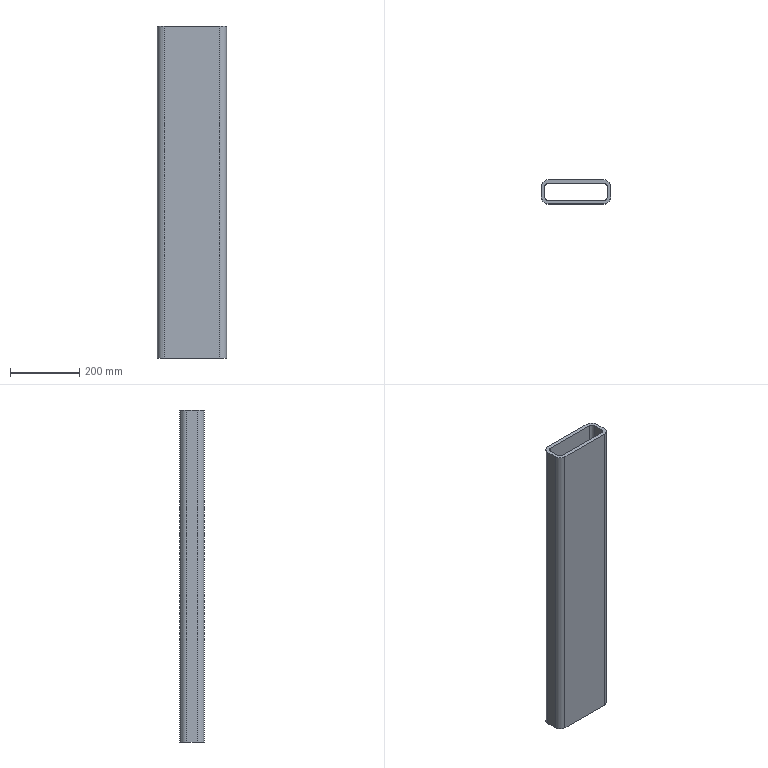Component | SolidWorks | Part12-1 | 1 solid | 18 faces | box 200 x 70 x 960 mm | volume 4552779 mm3 | plane 10 | cylinder 8 | commonest cylinder face diameters 40 x4 20 x4 | material Electroplated Steel
build123d program:
from build123d import *

# Parameters (mm, degrees)
BOSS_EXTRUDE1_DEPTH = 480


with BuildPart() as part:
    # Sketch1 → Boss-Extrude1 (new, symmetric)
    with BuildSketch(Plane.XY):
        with BuildLine():
            Line((80, -35), (-80, -35))
            ThreePointArc((-80, -35), (-94.142, -29.142), (-100, -15))
            Line((-100, -15), (-100, 15))
            ThreePointArc((-100, 15), (-94.142, 29.142), (-80, 35))
            Line((-80, 35), (80, 35))
            ThreePointArc((80, 35), (94.142, 29.142), (100, 15))
            Line((100, 15), (100, -15))
            ThreePointArc((100, -15), (94.142, -29.142), (80, -35))
        make_face()
        with BuildLine():
            Line((80, 25), (-80, 25))
            ThreePointArc((-80, 25), (-87.071, 22.071), (-90, 15))
            Line((-90, 15), (-90, -15))
            ThreePointArc((-90, -15), (-87.071, -22.071), (-80, -25))
            Line((-80, -25), (80, -25))
            ThreePointArc((80, -25), (87.071, -22.071), (90, -15))
            Line((90, -15), (90, 15))
            ThreePointArc((90, 15), (87.071, 22.071), (80, 25))
        make_face(mode=Mode.SUBTRACT)
    extrude(amount=BOSS_EXTRUDE1_DEPTH, both=True)


solid = part.part

# Placed as in the assembly
solid = solid.moved(Location((-7.456, -303.275, 860), (0, 0, 0)))
STEP:
#1=COLOUR_RGB('',0.7922,0.8196,0.9333);
#2=FILL_AREA_STYLE_COLOUR('',#1);
#3=FILL_AREA_STYLE('',(#2));
#4=SURFACE_STYLE_FILL_AREA(#3);
#5=SURFACE_SIDE_STYLE('',(#4));
#6=SURFACE_STYLE_USAGE(.BOTH.,#5);
#7=PRESENTATION_STYLE_ASSIGNMENT((#6));
#8=CARTESIAN_POINT('',(3.643,-12.531,14.961));
#9=VERTEX_POINT('',#8);
#10=CARTESIAN_POINT('',(2.856,-13.318,14.961));
#11=VERTEX_POINT('',#10);
#12=CARTESIAN_POINT('',(2.856,-12.531,14.961));
#13=DIRECTION('',(0.,0.,-1.));
#14=DIRECTION('',(1.,0.,0.));
#15=AXIS2_PLACEMENT_3D('',#12,#13,#14);
#16=CIRCLE('',#15,0.7874);
#17=EDGE_CURVE('',#9,#11,#16,.T.);
#18=ORIENTED_EDGE('',*,*,#17,.T.);
#19=CARTESIAN_POINT('',(-3.443,-13.318,14.961));
#20=VERTEX_POINT('',#19);
#21=CARTESIAN_POINT('',(-3.443,-13.318,14.961));
#22=DIRECTION('',(-1.,-0.,0.));
#23=VECTOR('',#22,39.37);
#24=LINE('',#21,#23);
#25=EDGE_CURVE('',#11,#20,#24,.T.);
#26=ORIENTED_EDGE('',*,*,#25,.T.);
#27=CARTESIAN_POINT('',(-4.231,-12.531,14.961));
#28=VERTEX_POINT('',#27);
#29=CARTESIAN_POINT('',(-3.443,-12.531,14.961));
#30=DIRECTION('',(0.,0.,-1.));
#31=DIRECTION('',(1.,0.,0.));
#32=AXIS2_PLACEMENT_3D('',#29,#30,#31);
#33=CIRCLE('',#32,0.7874);
#34=EDGE_CURVE('',#20,#28,#33,.T.);
#35=ORIENTED_EDGE('',*,*,#34,.T.);
#36=CARTESIAN_POINT('',(-4.231,-11.349,14.961));
#37=VERTEX_POINT('',#36);
#38=CARTESIAN_POINT('',(-4.231,-12.531,14.961));
#39=DIRECTION('',(-0.,1.,0.));
#40=VECTOR('',#39,39.37);
#41=LINE('',#38,#40);
#42=EDGE_CURVE('',#28,#37,#41,.T.);
#43=ORIENTED_EDGE('',*,*,#42,.T.);
#44=CARTESIAN_POINT('',(-3.443,-10.562,14.961));
#45=VERTEX_POINT('',#44);
#46=CARTESIAN_POINT('',(-3.443,-11.349,14.961));
#47=DIRECTION('',(0.,0.,-1.));
#48=DIRECTION('',(-1.,0.,0.));
#49=AXIS2_PLACEMENT_3D('',#46,#47,#48);
#50=CIRCLE('',#49,0.7874);
#51=EDGE_CURVE('',#37,#45,#50,.T.);
#52=ORIENTED_EDGE('',*,*,#51,.T.);
#53=CARTESIAN_POINT('',(2.856,-10.562,14.961));
#54=VERTEX_POINT('',#53);
#55=CARTESIAN_POINT('',(-3.443,-10.562,14.961));
#56=DIRECTION('',(1.,0.,0.));
#57=VECTOR('',#56,39.37);
#58=LINE('',#55,#57);
#59=EDGE_CURVE('',#45,#54,#58,.T.);
#60=ORIENTED_EDGE('',*,*,#59,.T.);
#61=CARTESIAN_POINT('',(3.643,-11.349,14.961));
#62=VERTEX_POINT('',#61);
#63=CARTESIAN_POINT('',(2.856,-11.349,14.961));
#64=DIRECTION('',(0.,0.,-1.));
#65=DIRECTION('',(1.,0.,0.));
#66=AXIS2_PLACEMENT_3D('',#63,#64,#65);
#67=CIRCLE('',#66,0.7874);
#68=EDGE_CURVE('',#54,#62,#67,.T.);
#69=ORIENTED_EDGE('',*,*,#68,.T.);
#70=CARTESIAN_POINT('',(3.643,-12.531,14.961));
#71=DIRECTION('',(0.,-1.,0.));
#72=VECTOR('',#71,39.37);
#73=LINE('',#70,#72);
#74=EDGE_CURVE('',#62,#9,#73,.T.);
#75=ORIENTED_EDGE('',*,*,#74,.T.);
#76=EDGE_LOOP('',(#18,#26,#35,#43,#52,#60,#69,#75));
#77=FACE_OUTER_BOUND('',#76,.T.);
#78=CARTESIAN_POINT('',(-3.837,-11.349,14.961));
#79=VERTEX_POINT('',#78);
#80=CARTESIAN_POINT('',(-3.443,-10.956,14.961));
#81=VERTEX_POINT('',#80);
#82=CARTESIAN_POINT('',(-3.443,-11.349,14.961));
#83=DIRECTION('',(0.,0.,-1.));
#84=DIRECTION('',(-1.,0.,0.));
#85=AXIS2_PLACEMENT_3D('',#82,#83,#84);
#86=CIRCLE('',#85,0.3937);
#87=EDGE_CURVE('',#79,#81,#86,.T.);
#88=ORIENTED_EDGE('',*,*,#87,.F.);
#89=CARTESIAN_POINT('',(-3.837,-12.531,14.961));
#90=VERTEX_POINT('',#89);
#91=CARTESIAN_POINT('',(-3.837,-12.531,14.961));
#92=DIRECTION('',(-0.,1.,0.));
#93=VECTOR('',#92,39.37);
#94=LINE('',#91,#93);
#95=EDGE_CURVE('',#90,#79,#94,.T.);
#96=ORIENTED_EDGE('',*,*,#95,.F.);
#97=CARTESIAN_POINT('',(-3.443,-12.924,14.961));
#98=VERTEX_POINT('',#97);
#99=CARTESIAN_POINT('',(-3.443,-12.531,14.961));
#100=DIRECTION('',(0.,0.,-1.));
#101=DIRECTION('',(1.,0.,0.));
#102=AXIS2_PLACEMENT_3D('',#99,#100,#101);
#103=CIRCLE('',#102,0.3937);
#104=EDGE_CURVE('',#98,#90,#103,.T.);
#105=ORIENTED_EDGE('',*,*,#104,.F.);
#106=CARTESIAN_POINT('',(2.856,-12.924,14.961));
#107=VERTEX_POINT('',#106);
#108=CARTESIAN_POINT('',(-3.443,-12.924,14.961));
#109=DIRECTION('',(-1.,-0.,0.));
#110=VECTOR('',#109,39.37);
#111=LINE('',#108,#110);
#112=EDGE_CURVE('',#107,#98,#111,.T.);
#113=ORIENTED_EDGE('',*,*,#112,.F.);
#114=CARTESIAN_POINT('',(3.25,-12.531,14.961));
#115=VERTEX_POINT('',#114);
#116=CARTESIAN_POINT('',(2.856,-12.531,14.961));
#117=DIRECTION('',(0.,0.,-1.));
#118=DIRECTION('',(1.,0.,0.));
#119=AXIS2_PLACEMENT_3D('',#116,#117,#118);
#120=CIRCLE('',#119,0.3937);
#121=EDGE_CURVE('',#115,#107,#120,.T.);
#122=ORIENTED_EDGE('',*,*,#121,.F.);
#123=CARTESIAN_POINT('',(3.25,-11.349,14.961));
#124=VERTEX_POINT('',#123);
#125=CARTESIAN_POINT('',(3.25,-12.531,14.961));
#126=DIRECTION('',(0.,-1.,0.));
#127=VECTOR('',#126,39.37);
#128=LINE('',#125,#127);
#129=EDGE_CURVE('',#124,#115,#128,.T.);
#130=ORIENTED_EDGE('',*,*,#129,.F.);
#131=CARTESIAN_POINT('',(2.856,-10.956,14.961));
#132=VERTEX_POINT('',#131);
#133=CARTESIAN_POINT('',(2.856,-11.349,14.961));
#134=DIRECTION('',(0.,0.,-1.));
#135=DIRECTION('',(1.,0.,0.));
#136=AXIS2_PLACEMENT_3D('',#133,#134,#135);
#137=CIRCLE('',#136,0.3937);
#138=EDGE_CURVE('',#132,#124,#137,.T.);
#139=ORIENTED_EDGE('',*,*,#138,.F.);
#140=CARTESIAN_POINT('',(-3.443,-10.956,14.961));
#141=DIRECTION('',(1.,0.,0.));
#142=VECTOR('',#141,39.37);
#143=LINE('',#140,#142);
#144=EDGE_CURVE('',#81,#132,#143,.T.);
#145=ORIENTED_EDGE('',*,*,#144,.F.);
#146=EDGE_LOOP('',(#88,#96,#105,#113,#122,#130,#139,#145));
#147=FACE_BOUND('',#146,.T.);
#148=CARTESIAN_POINT('',(2.856,-12.531,14.961));
#149=DIRECTION('',(0.,0.,1.));
#150=DIRECTION('',(1.,0.,0.));
#151=AXIS2_PLACEMENT_3D('',#148,#149,#150);
#152=PLANE('',#151);
#153=ADVANCED_FACE('',(#77,#147),#152,.F.);
#154=CARTESIAN_POINT('',(3.643,-12.531,52.756));
#155=VERTEX_POINT('',#154);
#156=CARTESIAN_POINT('',(2.856,-13.318,52.756));
#157=VERTEX_POINT('',#156);
#158=CARTESIAN_POINT('',(2.856,-12.531,52.756));
#159=DIRECTION('',(0.,0.,-1.));
#160=DIRECTION('',(1.,0.,0.));
#161=AXIS2_PLACEMENT_3D('',#158,#159,#160);
#162=CIRCLE('',#161,0.7874);
#163=EDGE_CURVE('',#155,#157,#162,.T.);
#164=ORIENTED_EDGE('',*,*,#163,.F.);
#165=CARTESIAN_POINT('',(3.643,-11.349,52.756));
#166=VERTEX_POINT('',#165);
#167=CARTESIAN_POINT('',(3.643,-12.531,52.756));
#168=DIRECTION('',(0.,-1.,0.));
#169=VECTOR('',#168,39.37);
#170=LINE('',#167,#169);
#171=EDGE_CURVE('',#166,#155,#170,.T.);
#172=ORIENTED_EDGE('',*,*,#171,.F.);
#173=CARTESIAN_POINT('',(2.856,-10.562,52.756));
#174=VERTEX_POINT('',#173);
#175=CARTESIAN_POINT('',(2.856,-11.349,52.756));
#176=DIRECTION('',(0.,0.,-1.));
#177=DIRECTION('',(1.,0.,0.));
#178=AXIS2_PLACEMENT_3D('',#175,#176,#177);
#179=CIRCLE('',#178,0.7874);
#180=EDGE_CURVE('',#174,#166,#179,.T.);
#181=ORIENTED_EDGE('',*,*,#180,.F.);
#182=CARTESIAN_POINT('',(-3.443,-10.562,52.756));
#183=VERTEX_POINT('',#182);
#184=CARTESIAN_POINT('',(-3.443,-10.562,52.756));
#185=DIRECTION('',(1.,0.,0.));
#186=VECTOR('',#185,39.37);
#187=LINE('',#184,#186);
#188=EDGE_CURVE('',#183,#174,#187,.T.);
#189=ORIENTED_EDGE('',*,*,#188,.F.);
#190=CARTESIAN_POINT('',(-4.231,-11.349,52.756));
#191=VERTEX_POINT('',#190);
#192=CARTESIAN_POINT('',(-3.443,-11.349,52.756));
#193=DIRECTION('',(0.,0.,-1.));
#194=DIRECTION('',(-1.,0.,0.));
#195=AXIS2_PLACEMENT_3D('',#192,#193,#194);
#196=CIRCLE('',#195,0.7874);
#197=EDGE_CURVE('',#191,#183,#196,.T.);
#198=ORIENTED_EDGE('',*,*,#197,.F.);
#199=CARTESIAN_POINT('',(-4.231,-12.531,52.756));
#200=VERTEX_POINT('',#199);
#201=CARTESIAN_POINT('',(-4.231,-12.531,52.756));
#202=DIRECTION('',(-0.,1.,0.));
#203=VECTOR('',#202,39.37);
#204=LINE('',#201,#203);
#205=EDGE_CURVE('',#200,#191,#204,.T.);
#206=ORIENTED_EDGE('',*,*,#205,.F.);
#207=CARTESIAN_POINT('',(-3.443,-13.318,52.756));
#208=VERTEX_POINT('',#207);
#209=CARTESIAN_POINT('',(-3.443,-12.531,52.756));
#210=DIRECTION('',(0.,0.,-1.));
#211=DIRECTION('',(1.,0.,0.));
#212=AXIS2_PLACEMENT_3D('',#209,#210,#211);
#213=CIRCLE('',#212,0.7874);
#214=EDGE_CURVE('',#208,#200,#213,.T.);
#215=ORIENTED_EDGE('',*,*,#214,.F.);
#216=CARTESIAN_POINT('',(-3.443,-13.318,52.756));
#217=DIRECTION('',(-1.,-0.,0.));
#218=VECTOR('',#217,39.37);
#219=LINE('',#216,#218);
#220=EDGE_CURVE('',#157,#208,#219,.T.);
#221=ORIENTED_EDGE('',*,*,#220,.F.);
#222=EDGE_LOOP('',(#164,#172,#181,#189,#198,#206,#215,#221));
#223=FACE_OUTER_BOUND('',#222,.T.);
#224=CARTESIAN_POINT('',(-3.837,-12.531,52.756));
#225=VERTEX_POINT('',#224);
#226=CARTESIAN_POINT('',(-3.837,-11.349,52.756));
#227=VERTEX_POINT('',#226);
#228=CARTESIAN_POINT('',(-3.837,-12.531,52.756));
#229=DIRECTION('',(-0.,1.,0.));
#230=VECTOR('',#229,39.37);
#231=LINE('',#228,#230);
#232=EDGE_CURVE('',#225,#227,#231,.T.);
#233=ORIENTED_EDGE('',*,*,#232,.T.);
#234=CARTESIAN_POINT('',(-3.443,-10.956,52.756));
#235=VERTEX_POINT('',#234);
#236=CARTESIAN_POINT('',(-3.443,-11.349,52.756));
#237=DIRECTION('',(0.,0.,-1.));
#238=DIRECTION('',(-1.,0.,0.));
#239=AXIS2_PLACEMENT_3D('',#236,#237,#238);
#240=CIRCLE('',#239,0.3937);
#241=EDGE_CURVE('',#227,#235,#240,.T.);
#242=ORIENTED_EDGE('',*,*,#241,.T.);
#243=CARTESIAN_POINT('',(2.856,-10.956,52.756));
#244=VERTEX_POINT('',#243);
#245=CARTESIAN_POINT('',(-3.443,-10.956,52.756));
#246=DIRECTION('',(1.,0.,0.));
#247=VECTOR('',#246,39.37);
#248=LINE('',#245,#247);
#249=EDGE_CURVE('',#235,#244,#248,.T.);
#250=ORIENTED_EDGE('',*,*,#249,.T.);
#251=CARTESIAN_POINT('',(3.25,-11.349,52.756));
#252=VERTEX_POINT('',#251);
#253=CARTESIAN_POINT('',(2.856,-11.349,52.756));
#254=DIRECTION('',(0.,0.,-1.));
#255=DIRECTION('',(1.,0.,0.));
#256=AXIS2_PLACEMENT_3D('',#253,#254,#255);
#257=CIRCLE('',#256,0.3937);
#258=EDGE_CURVE('',#244,#252,#257,.T.);
#259=ORIENTED_EDGE('',*,*,#258,.T.);
#260=CARTESIAN_POINT('',(3.25,-12.531,52.756));
#261=VERTEX_POINT('',#260);
#262=CARTESIAN_POINT('',(3.25,-12.531,52.756));
#263=DIRECTION('',(0.,-1.,0.));
#264=VECTOR('',#263,39.37);
#265=LINE('',#262,#264);
#266=EDGE_CURVE('',#252,#261,#265,.T.);
#267=ORIENTED_EDGE('',*,*,#266,.T.);
#268=CARTESIAN_POINT('',(2.856,-12.924,52.756));
#269=VERTEX_POINT('',#268);
#270=CARTESIAN_POINT('',(2.856,-12.531,52.756));
#271=DIRECTION('',(0.,0.,-1.));
#272=DIRECTION('',(1.,0.,0.));
#273=AXIS2_PLACEMENT_3D('',#270,#271,#272);
#274=CIRCLE('',#273,0.3937);
#275=EDGE_CURVE('',#261,#269,#274,.T.);
#276=ORIENTED_EDGE('',*,*,#275,.T.);
#277=CARTESIAN_POINT('',(-3.443,-12.924,52.756));
#278=VERTEX_POINT('',#277);
#279=CARTESIAN_POINT('',(-3.443,-12.924,52.756));
#280=DIRECTION('',(-1.,-0.,0.));
#281=VECTOR('',#280,39.37);
#282=LINE('',#279,#281);
#283=EDGE_CURVE('',#269,#278,#282,.T.);
#284=ORIENTED_EDGE('',*,*,#283,.T.);
#285=CARTESIAN_POINT('',(-3.443,-12.531,52.756));
#286=DIRECTION('',(0.,0.,-1.));
#287=DIRECTION('',(1.,0.,0.));
#288=AXIS2_PLACEMENT_3D('',#285,#286,#287);
#289=CIRCLE('',#288,0.3937);
#290=EDGE_CURVE('',#278,#225,#289,.T.);
#291=ORIENTED_EDGE('',*,*,#290,.T.);
#292=EDGE_LOOP('',(#233,#242,#250,#259,#267,#276,#284,#291));
#293=FACE_BOUND('',#292,.T.);
#294=CARTESIAN_POINT('',(2.856,-12.531,52.756));
#295=DIRECTION('',(0.,0.,1.));
#296=DIRECTION('',(1.,0.,0.));
#297=AXIS2_PLACEMENT_3D('',#294,#295,#296);
#298=PLANE('',#297);
#299=ADVANCED_FACE('',(#223,#293),#298,.T.);
#300=ORIENTED_EDGE('',*,*,#163,.T.);
#301=CARTESIAN_POINT('',(2.856,-13.318,14.961));
#302=DIRECTION('',(0.,0.,1.));
#303=VECTOR('',#302,39.37);
#304=LINE('',#301,#303);
#305=EDGE_CURVE('',#11,#157,#304,.T.);
#306=ORIENTED_EDGE('',*,*,#305,.F.);
#307=ORIENTED_EDGE('',*,*,#17,.F.);
#308=CARTESIAN_POINT('',(3.643,-12.531,14.961));
#309=DIRECTION('',(0.,0.,1.));
#310=VECTOR('',#309,39.37);
#311=LINE('',#308,#310);
#312=EDGE_CURVE('',#9,#155,#311,.T.);
#313=ORIENTED_EDGE('',*,*,#312,.T.);
#314=EDGE_LOOP('',(#300,#306,#307,#313));
#315=FACE_OUTER_BOUND('',#314,.T.);
#316=CARTESIAN_POINT('',(2.856,-12.531,14.961));
#317=DIRECTION('',(0.,0.,1.));
#318=DIRECTION('',(1.,0.,0.));
#319=AXIS2_PLACEMENT_3D('',#316,#317,#318);
#320=CYLINDRICAL_SURFACE('',#319,0.7874);
#321=ADVANCED_FACE('',(#315),#320,.T.);
#322=ORIENTED_EDGE('',*,*,#220,.T.);
#323=CARTESIAN_POINT('',(-3.443,-13.318,14.961));
#324=DIRECTION('',(0.,0.,1.));
#325=VECTOR('',#324,39.37);
#326=LINE('',#323,#325);
#327=EDGE_CURVE('',#20,#208,#326,.T.);
#328=ORIENTED_EDGE('',*,*,#327,.F.);
#329=ORIENTED_EDGE('',*,*,#25,.F.);
#330=ORIENTED_EDGE('',*,*,#305,.T.);
#331=EDGE_LOOP('',(#322,#328,#329,#330));
#332=FACE_OUTER_BOUND('',#331,.T.);
#333=CARTESIAN_POINT('',(-3.443,-13.318,14.961));
#334=DIRECTION('',(-0.,1.,0.));
#335=DIRECTION('',(1.,0.,0.));
#336=AXIS2_PLACEMENT_3D('',#333,#334,#335);
#337=PLANE('',#336);
#338=ADVANCED_FACE('',(#332),#337,.F.);
#339=ORIENTED_EDGE('',*,*,#214,.T.);
#340=CARTESIAN_POINT('',(-4.231,-12.531,14.961));
#341=DIRECTION('',(0.,0.,1.));
#342=VECTOR('',#341,39.37);
#343=LINE('',#340,#342);
#344=EDGE_CURVE('',#28,#200,#343,.T.);
#345=ORIENTED_EDGE('',*,*,#344,.F.);
#346=ORIENTED_EDGE('',*,*,#34,.F.);
#347=ORIENTED_EDGE('',*,*,#327,.T.);
#348=EDGE_LOOP('',(#339,#345,#346,#347));
#349=FACE_OUTER_BOUND('',#348,.T.);
#350=CARTESIAN_POINT('',(-3.443,-12.531,14.961));
#351=DIRECTION('',(0.,0.,1.));
#352=DIRECTION('',(1.,0.,0.));
#353=AXIS2_PLACEMENT_3D('',#350,#351,#352);
#354=CYLINDRICAL_SURFACE('',#353,0.7874);
#355=ADVANCED_FACE('',(#349),#354,.T.);
#356=ORIENTED_EDGE('',*,*,#205,.T.);
#357=CARTESIAN_POINT('',(-4.231,-11.349,14.961));
#358=DIRECTION('',(0.,0.,1.));
#359=VECTOR('',#358,39.37);
#360=LINE('',#357,#359);
#361=EDGE_CURVE('',#37,#191,#360,.T.);
#362=ORIENTED_EDGE('',*,*,#361,.F.);
#363=ORIENTED_EDGE('',*,*,#42,.F.);
#364=ORIENTED_EDGE('',*,*,#344,.T.);
#365=EDGE_LOOP('',(#356,#362,#363,#364));
#366=FACE_OUTER_BOUND('',#365,.T.);
#367=CARTESIAN_POINT('',(-4.231,-12.531,14.961));
#368=DIRECTION('',(1.,0.,0.));
#369=DIRECTION('',(0.,0.,-1.));
#370=AXIS2_PLACEMENT_3D('',#367,#368,#369);
#371=PLANE('',#370);
#372=ADVANCED_FACE('',(#366),#371,.F.);
#373=ORIENTED_EDGE('',*,*,#197,.T.);
#374=CARTESIAN_POINT('',(-3.443,-10.562,14.961));
#375=DIRECTION('',(0.,0.,1.));
#376=VECTOR('',#375,39.37);
#377=LINE('',#374,#376);
#378=EDGE_CURVE('',#45,#183,#377,.T.);
#379=ORIENTED_EDGE('',*,*,#378,.F.);
#380=ORIENTED_EDGE('',*,*,#51,.F.);
#381=ORIENTED_EDGE('',*,*,#361,.T.);
#382=EDGE_LOOP('',(#373,#379,#380,#381));
#383=FACE_OUTER_BOUND('',#382,.T.);
#384=CARTESIAN_POINT('',(-3.443,-11.349,14.961));
#385=DIRECTION('',(0.,0.,1.));
#386=DIRECTION('',(1.,0.,0.));
#387=AXIS2_PLACEMENT_3D('',#384,#385,#386);
#388=CYLINDRICAL_SURFACE('',#387,0.7874);
#389=ADVANCED_FACE('',(#383),#388,.T.);
#390=ORIENTED_EDGE('',*,*,#188,.T.);
#391=CARTESIAN_POINT('',(2.856,-10.562,14.961));
#392=DIRECTION('',(0.,0.,1.));
#393=VECTOR('',#392,39.37);
#394=LINE('',#391,#393);
#395=EDGE_CURVE('',#54,#174,#394,.T.);
#396=ORIENTED_EDGE('',*,*,#395,.F.);
#397=ORIENTED_EDGE('',*,*,#59,.F.);
#398=ORIENTED_EDGE('',*,*,#378,.T.);
#399=EDGE_LOOP('',(#390,#396,#397,#398));
#400=FACE_OUTER_BOUND('',#399,.T.);
#401=CARTESIAN_POINT('',(-3.443,-10.562,14.961));
#402=DIRECTION('',(0.,-1.,0.));
#403=DIRECTION('',(-1.,-0.,0.));
#404=AXIS2_PLACEMENT_3D('',#401,#402,#403);
#405=PLANE('',#404);
#406=ADVANCED_FACE('',(#400),#405,.F.);
#407=ORIENTED_EDGE('',*,*,#180,.T.);
#408=CARTESIAN_POINT('',(3.643,-11.349,14.961));
#409=DIRECTION('',(0.,0.,1.));
#410=VECTOR('',#409,39.37);
#411=LINE('',#408,#410);
#412=EDGE_CURVE('',#62,#166,#411,.T.);
#413=ORIENTED_EDGE('',*,*,#412,.F.);
#414=ORIENTED_EDGE('',*,*,#68,.F.);
#415=ORIENTED_EDGE('',*,*,#395,.T.);
#416=EDGE_LOOP('',(#407,#413,#414,#415));
#417=FACE_OUTER_BOUND('',#416,.T.);
#418=CARTESIAN_POINT('',(2.856,-11.349,14.961));
#419=DIRECTION('',(0.,0.,1.));
#420=DIRECTION('',(1.,0.,0.));
#421=AXIS2_PLACEMENT_3D('',#418,#419,#420);
#422=CYLINDRICAL_SURFACE('',#421,0.7874);
#423=ADVANCED_FACE('',(#417),#422,.T.);
#424=ORIENTED_EDGE('',*,*,#171,.T.);
#425=ORIENTED_EDGE('',*,*,#312,.F.);
#426=ORIENTED_EDGE('',*,*,#74,.F.);
#427=ORIENTED_EDGE('',*,*,#412,.T.);
#428=EDGE_LOOP('',(#424,#425,#426,#427));
#429=FACE_OUTER_BOUND('',#428,.T.);
#430=CARTESIAN_POINT('',(3.643,-12.531,14.961));
#431=DIRECTION('',(-1.,-0.,0.));
#432=DIRECTION('',(0.,0.,1.));
#433=AXIS2_PLACEMENT_3D('',#430,#431,#432);
#434=PLANE('',#433);
#435=ADVANCED_FACE('',(#429),#434,.F.);
#436=ORIENTED_EDGE('',*,*,#241,.F.);
#437=CARTESIAN_POINT('',(-3.837,-11.349,14.961));
#438=DIRECTION('',(0.,0.,1.));
#439=VECTOR('',#438,39.37);
#440=LINE('',#437,#439);
#441=EDGE_CURVE('',#79,#227,#440,.T.);
#442=ORIENTED_EDGE('',*,*,#441,.F.);
#443=ORIENTED_EDGE('',*,*,#87,.T.);
#444=CARTESIAN_POINT('',(-3.443,-10.956,14.961));
#445=DIRECTION('',(0.,0.,1.));
#446=VECTOR('',#445,39.37);
#447=LINE('',#444,#446);
#448=EDGE_CURVE('',#81,#235,#447,.T.);
#449=ORIENTED_EDGE('',*,*,#448,.T.);
#450=EDGE_LOOP('',(#436,#442,#443,#449));
#451=FACE_OUTER_BOUND('',#450,.T.);
#452=CARTESIAN_POINT('',(-3.443,-11.349,14.961));
#453=DIRECTION('',(0.,0.,1.));
#454=DIRECTION('',(1.,0.,0.));
#455=AXIS2_PLACEMENT_3D('',#452,#453,#454);
#456=CYLINDRICAL_SURFACE('',#455,0.3937);
#457=ADVANCED_FACE('',(#451),#456,.F.);
#458=ORIENTED_EDGE('',*,*,#249,.F.);
#459=ORIENTED_EDGE('',*,*,#448,.F.);
#460=ORIENTED_EDGE('',*,*,#144,.T.);
#461=CARTESIAN_POINT('',(2.856,-10.956,14.961));
#462=DIRECTION('',(0.,0.,1.));
#463=VECTOR('',#462,39.37);
#464=LINE('',#461,#463);
#465=EDGE_CURVE('',#132,#244,#464,.T.);
#466=ORIENTED_EDGE('',*,*,#465,.T.);
#467=EDGE_LOOP('',(#458,#459,#460,#466));
#468=FACE_OUTER_BOUND('',#467,.T.);
#469=CARTESIAN_POINT('',(-3.443,-10.956,14.961));
#470=DIRECTION('',(0.,-1.,0.));
#471=DIRECTION('',(-1.,-0.,0.));
#472=AXIS2_PLACEMENT_3D('',#469,#470,#471);
#473=PLANE('',#472);
#474=ADVANCED_FACE('',(#468),#473,.T.);
#475=ORIENTED_EDGE('',*,*,#258,.F.);
#476=ORIENTED_EDGE('',*,*,#465,.F.);
#477=ORIENTED_EDGE('',*,*,#138,.T.);
#478=CARTESIAN_POINT('',(3.25,-11.349,14.961));
#479=DIRECTION('',(0.,0.,1.));
#480=VECTOR('',#479,39.37);
#481=LINE('',#478,#480);
#482=EDGE_CURVE('',#124,#252,#481,.T.);
#483=ORIENTED_EDGE('',*,*,#482,.T.);
#484=EDGE_LOOP('',(#475,#476,#477,#483));
#485=FACE_OUTER_BOUND('',#484,.T.);
#486=CARTESIAN_POINT('',(2.856,-11.349,14.961));
#487=DIRECTION('',(0.,0.,1.));
#488=DIRECTION('',(1.,0.,0.));
#489=AXIS2_PLACEMENT_3D('',#486,#487,#488);
#490=CYLINDRICAL_SURFACE('',#489,0.3937);
#491=ADVANCED_FACE('',(#485),#490,.F.);
#492=ORIENTED_EDGE('',*,*,#266,.F.);
#493=ORIENTED_EDGE('',*,*,#482,.F.);
#494=ORIENTED_EDGE('',*,*,#129,.T.);
#495=CARTESIAN_POINT('',(3.25,-12.531,14.961));
#496=DIRECTION('',(0.,0.,1.));
#497=VECTOR('',#496,39.37);
#498=LINE('',#495,#497);
#499=EDGE_CURVE('',#115,#261,#498,.T.);
#500=ORIENTED_EDGE('',*,*,#499,.T.);
#501=EDGE_LOOP('',(#492,#493,#494,#500));
#502=FACE_OUTER_BOUND('',#501,.T.);
#503=CARTESIAN_POINT('',(3.25,-12.531,14.961));
#504=DIRECTION('',(-1.,-0.,0.));
#505=DIRECTION('',(0.,0.,1.));
#506=AXIS2_PLACEMENT_3D('',#503,#504,#505);
#507=PLANE('',#506);
#508=ADVANCED_FACE('',(#502),#507,.T.);
#509=ORIENTED_EDGE('',*,*,#275,.F.);
#510=ORIENTED_EDGE('',*,*,#499,.F.);
#511=ORIENTED_EDGE('',*,*,#121,.T.);
#512=CARTESIAN_POINT('',(2.856,-12.924,14.961));
#513=DIRECTION('',(0.,0.,1.));
#514=VECTOR('',#513,39.37);
#515=LINE('',#512,#514);
#516=EDGE_CURVE('',#107,#269,#515,.T.);
#517=ORIENTED_EDGE('',*,*,#516,.T.);
#518=EDGE_LOOP('',(#509,#510,#511,#517));
#519=FACE_OUTER_BOUND('',#518,.T.);
#520=CARTESIAN_POINT('',(2.856,-12.531,14.961));
#521=DIRECTION('',(0.,0.,1.));
#522=DIRECTION('',(1.,0.,0.));
#523=AXIS2_PLACEMENT_3D('',#520,#521,#522);
#524=CYLINDRICAL_SURFACE('',#523,0.3937);
#525=ADVANCED_FACE('',(#519),#524,.F.);
#526=ORIENTED_EDGE('',*,*,#283,.F.);
#527=ORIENTED_EDGE('',*,*,#516,.F.);
#528=ORIENTED_EDGE('',*,*,#112,.T.);
#529=CARTESIAN_POINT('',(-3.443,-12.924,14.961));
#530=DIRECTION('',(0.,0.,1.));
#531=VECTOR('',#530,39.37);
#532=LINE('',#529,#531);
#533=EDGE_CURVE('',#98,#278,#532,.T.);
#534=ORIENTED_EDGE('',*,*,#533,.T.);
#535=EDGE_LOOP('',(#526,#527,#528,#534));
#536=FACE_OUTER_BOUND('',#535,.T.);
#537=CARTESIAN_POINT('',(-3.443,-12.924,14.961));
#538=DIRECTION('',(-0.,1.,0.));
#539=DIRECTION('',(1.,0.,0.));
#540=AXIS2_PLACEMENT_3D('',#537,#538,#539);
#541=PLANE('',#540);
#542=ADVANCED_FACE('',(#536),#541,.T.);
#543=ORIENTED_EDGE('',*,*,#290,.F.);
#544=ORIENTED_EDGE('',*,*,#533,.F.);
#545=ORIENTED_EDGE('',*,*,#104,.T.);
#546=CARTESIAN_POINT('',(-3.837,-12.531,14.961));
#547=DIRECTION('',(0.,0.,1.));
#548=VECTOR('',#547,39.37);
#549=LINE('',#546,#548);
#550=EDGE_CURVE('',#90,#225,#549,.T.);
#551=ORIENTED_EDGE('',*,*,#550,.T.);
#552=EDGE_LOOP('',(#543,#544,#545,#551));
#553=FACE_OUTER_BOUND('',#552,.T.);
#554=CARTESIAN_POINT('',(-3.443,-12.531,14.961));
#555=DIRECTION('',(0.,0.,1.));
#556=DIRECTION('',(1.,0.,0.));
#557=AXIS2_PLACEMENT_3D('',#554,#555,#556);
#558=CYLINDRICAL_SURFACE('',#557,0.3937);
#559=ADVANCED_FACE('',(#553),#558,.F.);
#560=ORIENTED_EDGE('',*,*,#232,.F.);
#561=ORIENTED_EDGE('',*,*,#550,.F.);
#562=ORIENTED_EDGE('',*,*,#95,.T.);
#563=ORIENTED_EDGE('',*,*,#441,.T.);
#564=EDGE_LOOP('',(#560,#561,#562,#563));
#565=FACE_OUTER_BOUND('',#564,.T.);
#566=CARTESIAN_POINT('',(-3.837,-12.531,14.961));
#567=DIRECTION('',(1.,0.,0.));
#568=DIRECTION('',(0.,-1.,0.));
#569=AXIS2_PLACEMENT_3D('',#566,#567,#568);
#570=PLANE('',#569);
#571=ADVANCED_FACE('',(#565),#570,.T.);
#572=CLOSED_SHELL('',(#153,#299,#321,#338,#355,#372,#389,#406,#423,#435,#457,#474,#491,#508,#525,#542,#559,#571));
#573=MANIFOLD_SOLID_BREP('',#572);
#574=STYLED_ITEM('',(#7),#573);
#575=PRESENTATION_LAYER_ASSIGNMENT('','',(#574));
#576=CARTESIAN_POINT('',(0.,0.,0.));
#577=DIRECTION('',(0.,0.,1.));
#578=DIRECTION('',(1.,0.,0.));
#579=AXIS2_PLACEMENT_3D('',#576,#577,#578);
#580=(LENGTH_UNIT()NAMED_UNIT(*)SI_UNIT($,.METRE.));
#581=LENGTH_MEASURE_WITH_UNIT(LENGTH_MEASURE(0.0254),#580);
#582=DIMENSIONAL_EXPONENTS(1.,0.,0.,0.,0.,0.,0.);
#583=(CONVERSION_BASED_UNIT('',#581)LENGTH_UNIT()NAMED_UNIT(#582));
#584=UNCERTAINTY_MEASURE_WITH_UNIT(LENGTH_MEASURE(0.00001),#583,'','');
#585=(NAMED_UNIT(*)PLANE_ANGLE_UNIT()SI_UNIT($,.RADIAN.));
#586=(NAMED_UNIT(*)SI_UNIT($,.STERADIAN.)SOLID_ANGLE_UNIT());
#587=(GEOMETRIC_REPRESENTATION_CONTEXT(3)GLOBAL_UNCERTAINTY_ASSIGNED_CONTEXT((#584))GLOBAL_UNIT_ASSIGNED_CONTEXT((#583,#585,#586))REPRESENTATION_CONTEXT('',''));
#588=ADVANCED_BREP_SHAPE_REPRESENTATION('',(#573,#579),#587);
#589=(LENGTH_UNIT()NAMED_UNIT(*)SI_UNIT($,.METRE.));
#590=LENGTH_MEASURE_WITH_UNIT(LENGTH_MEASURE(0.0254),#589);
#591=DIMENSIONAL_EXPONENTS(1.,0.,0.,0.,0.,0.,0.);
#592=(CONVERSION_BASED_UNIT('',#590)LENGTH_UNIT()NAMED_UNIT(#591));
#593=UNCERTAINTY_MEASURE_WITH_UNIT(LENGTH_MEASURE(0.00001),#592,'','');
#594=(NAMED_UNIT(*)PLANE_ANGLE_UNIT()SI_UNIT($,.RADIAN.));
#595=(NAMED_UNIT(*)SI_UNIT($,.STERADIAN.)SOLID_ANGLE_UNIT());
#596=(GEOMETRIC_REPRESENTATION_CONTEXT(3)GLOBAL_UNCERTAINTY_ASSIGNED_CONTEXT((#593))GLOBAL_UNIT_ASSIGNED_CONTEXT((#592,#594,#595))REPRESENTATION_CONTEXT('',''));
#597=MECHANICAL_DESIGN_GEOMETRIC_PRESENTATION_REPRESENTATION('',(#574),#596);